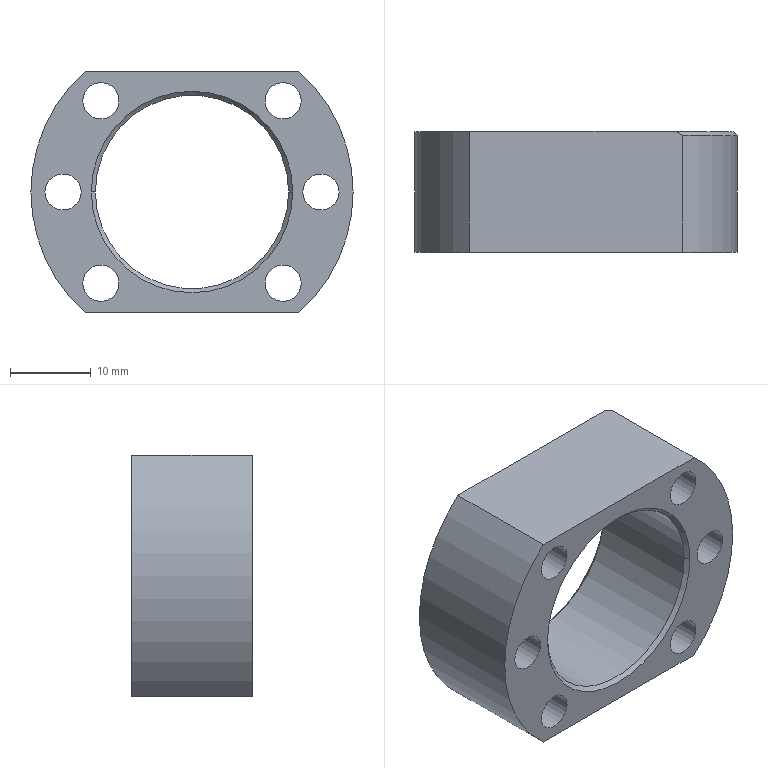Component | SolidWorks | F01AE00111-A2085-1 | 1 solid | 27 faces | box 40 x 15 x 30 mm | volume 7889 mm3 | cylinder 17 | cone 6 | plane 4 | commonest cylinder face diameters 4.5 x12 40 x3 24 x2 | material 6061 Alloy
build123d program:
from build123d import *

# Parameters (mm, degrees)
SKETCH1_R                  = 20
SKETCH1_R_2                = 12
BOSS_EXTRUDE1_DEPTH        = 15
CUT_EXTRUDE1_DEPTH         = 33.016
CHAMFER1_SIZE              = 0.5
F_4_5_4_5_DIAMETER_HOLE1_D = 4.5


with BuildPart() as part:
    # Sketch1 → Boss-Extrude1 (new body)
    with BuildSketch(Plane(origin=(0, 0, 0), x_dir=(1, 0, 0), z_dir=(0, 1, 0))):
        with Locations(Location((0, 0, 0), (0, 0, 270))):
            Circle(SKETCH1_R)
        with Locations(Location((0, 0, 0), (0, 0, 270))):
            Circle(SKETCH1_R_2, mode=Mode.SUBTRACT)
    extrude(amount=BOSS_EXTRUDE1_DEPTH)

    # Sketch2 → Cut-Extrude1 (cut, symmetric)
    with BuildSketch(Plane(origin=(0, 15, 0), x_dir=(1, 0, 0), z_dir=(0, 1, 0))):
        Polygon((15, 119.751), (15, 13.229), (15, -13.229), (15, -119.751), (228.045, -119.751), (228.045, 119.751), align=None)
    cut_extrude1 = extrude(amount=CUT_EXTRUDE1_DEPTH, both=True, mode=Mode.SUBTRACT)

    # Mirror1: Cut-Extrude1 across plane
    add(cut_extrude1.mirror(Plane(origin=(0, 0, 0), x_dir=(0, 0, 1), z_dir=(1, 0, 0))), mode=Mode.SUBTRACT)

    # Chamfer1
    chamfer1_edges = [part.edges().sort_by_distance(p)[0] for p in [
        (0, 0, -12),
        (0, 15, -12),
        (0, 15, -20),
    ]]
    chamfer(chamfer1_edges, length=CHAMFER1_SIZE)

    # 4.5 _4.5_ Diameter Hole1 (through all)
    with Locations(Plane(origin=(0, 15, 0), x_dir=(1, 0, 0), z_dir=(0, 1, 0))):
        with Locations((-11.314, 11.314), (0, 16), (11.314, 11.314), (-11.314, -11.314), (0, -16), (11.314, -11.314)):
            Hole(F_4_5_4_5_DIAMETER_HOLE1_D / 2)


solid = part.part

# Placed as in the assembly
solid = solid.moved(Location((-109.352, -190.452, -272.475), (0, -90, 0)))
STEP:
#1=CARTESIAN_POINT('',(-3.771,-7.498,-11.173));
#2=VERTEX_POINT('',#1);
#3=CARTESIAN_POINT('',(-3.948,-7.498,-11.173));
#4=VERTEX_POINT('',#3);
#5=CARTESIAN_POINT('',(-3.86,-7.498,-11.173));
#6=DIRECTION('',(-0.,1.,0.));
#7=DIRECTION('',(-1.,0.,0.));
#8=AXIS2_PLACEMENT_3D('',#5,#6,#7);
#9=CIRCLE('',#8,0.08858);
#10=EDGE_CURVE('',#2,#4,#9,.T.);
#11=ORIENTED_EDGE('',*,*,#10,.F.);
#12=CARTESIAN_POINT('',(-3.771,-6.908,-11.173));
#13=VERTEX_POINT('',#12);
#14=CARTESIAN_POINT('',(-3.771,-6.908,-11.173));
#15=DIRECTION('',(-0.,1.,0.));
#16=VECTOR('',#15,39.37);
#17=LINE('',#14,#16);
#18=EDGE_CURVE('',#2,#13,#17,.T.);
#19=ORIENTED_EDGE('',*,*,#18,.T.);
#20=CARTESIAN_POINT('',(-3.948,-6.908,-11.173));
#21=VERTEX_POINT('',#20);
#22=CARTESIAN_POINT('',(-3.86,-6.908,-11.173));
#23=DIRECTION('',(-0.,1.,0.));
#24=DIRECTION('',(-1.,0.,0.));
#25=AXIS2_PLACEMENT_3D('',#22,#23,#24);
#26=CIRCLE('',#25,0.08858);
#27=EDGE_CURVE('',#13,#21,#26,.T.);
#28=ORIENTED_EDGE('',*,*,#27,.T.);
#29=CARTESIAN_POINT('',(-3.948,-6.908,-11.173));
#30=DIRECTION('',(-0.,1.,0.));
#31=VECTOR('',#30,39.37);
#32=LINE('',#29,#31);
#33=EDGE_CURVE('',#4,#21,#32,.T.);
#34=ORIENTED_EDGE('',*,*,#33,.F.);
#35=EDGE_LOOP('',(#11,#19,#28,#34));
#36=FACE_OUTER_BOUND('',#35,.T.);
#37=CARTESIAN_POINT('',(-3.86,-6.908,-11.173));
#38=DIRECTION('',(-0.,1.,0.));
#39=DIRECTION('',(-1.,0.,0.));
#40=AXIS2_PLACEMENT_3D('',#37,#38,#39);
#41=CYLINDRICAL_SURFACE('',#40,0.08858);
#42=ADVANCED_FACE('',(#36),#41,.F.);
#43=CARTESIAN_POINT('',(-3.587,-7.498,-10.727));
#44=VERTEX_POINT('',#43);
#45=CARTESIAN_POINT('',(-3.764,-7.498,-10.727));
#46=VERTEX_POINT('',#45);
#47=CARTESIAN_POINT('',(-3.675,-7.498,-10.727));
#48=DIRECTION('',(-0.,1.,0.));
#49=DIRECTION('',(-1.,0.,0.));
#50=AXIS2_PLACEMENT_3D('',#47,#48,#49);
#51=CIRCLE('',#50,0.08858);
#52=EDGE_CURVE('',#44,#46,#51,.T.);
#53=ORIENTED_EDGE('',*,*,#52,.F.);
#54=CARTESIAN_POINT('',(-3.587,-6.908,-10.727));
#55=VERTEX_POINT('',#54);
#56=CARTESIAN_POINT('',(-3.587,-6.908,-10.727));
#57=DIRECTION('',(-0.,1.,0.));
#58=VECTOR('',#57,39.37);
#59=LINE('',#56,#58);
#60=EDGE_CURVE('',#44,#55,#59,.T.);
#61=ORIENTED_EDGE('',*,*,#60,.T.);
#62=CARTESIAN_POINT('',(-3.764,-6.908,-10.727));
#63=VERTEX_POINT('',#62);
#64=CARTESIAN_POINT('',(-3.675,-6.908,-10.727));
#65=DIRECTION('',(-0.,1.,0.));
#66=DIRECTION('',(-1.,0.,0.));
#67=AXIS2_PLACEMENT_3D('',#64,#65,#66);
#68=CIRCLE('',#67,0.08858);
#69=EDGE_CURVE('',#55,#63,#68,.T.);
#70=ORIENTED_EDGE('',*,*,#69,.T.);
#71=CARTESIAN_POINT('',(-3.764,-6.908,-10.727));
#72=DIRECTION('',(-0.,1.,0.));
#73=VECTOR('',#72,39.37);
#74=LINE('',#71,#73);
#75=EDGE_CURVE('',#46,#63,#74,.T.);
#76=ORIENTED_EDGE('',*,*,#75,.F.);
#77=EDGE_LOOP('',(#53,#61,#70,#76));
#78=FACE_OUTER_BOUND('',#77,.T.);
#79=CARTESIAN_POINT('',(-3.675,-6.908,-10.727));
#80=DIRECTION('',(-0.,1.,0.));
#81=DIRECTION('',(-1.,0.,0.));
#82=AXIS2_PLACEMENT_3D('',#79,#80,#81);
#83=CYLINDRICAL_SURFACE('',#82,0.08858);
#84=ADVANCED_FACE('',(#78),#83,.F.);
#85=CARTESIAN_POINT('',(-3.771,-7.498,-10.282));
#86=VERTEX_POINT('',#85);
#87=CARTESIAN_POINT('',(-3.948,-7.498,-10.282));
#88=VERTEX_POINT('',#87);
#89=CARTESIAN_POINT('',(-3.86,-7.498,-10.282));
#90=DIRECTION('',(-0.,1.,0.));
#91=DIRECTION('',(-1.,0.,0.));
#92=AXIS2_PLACEMENT_3D('',#89,#90,#91);
#93=CIRCLE('',#92,0.08858);
#94=EDGE_CURVE('',#86,#88,#93,.T.);
#95=ORIENTED_EDGE('',*,*,#94,.F.);
#96=CARTESIAN_POINT('',(-3.771,-6.908,-10.282));
#97=VERTEX_POINT('',#96);
#98=CARTESIAN_POINT('',(-3.771,-6.908,-10.282));
#99=DIRECTION('',(-0.,1.,0.));
#100=VECTOR('',#99,39.37);
#101=LINE('',#98,#100);
#102=EDGE_CURVE('',#86,#97,#101,.T.);
#103=ORIENTED_EDGE('',*,*,#102,.T.);
#104=CARTESIAN_POINT('',(-3.948,-6.908,-10.282));
#105=VERTEX_POINT('',#104);
#106=CARTESIAN_POINT('',(-3.86,-6.908,-10.282));
#107=DIRECTION('',(-0.,1.,0.));
#108=DIRECTION('',(-1.,0.,0.));
#109=AXIS2_PLACEMENT_3D('',#106,#107,#108);
#110=CIRCLE('',#109,0.08858);
#111=EDGE_CURVE('',#97,#105,#110,.T.);
#112=ORIENTED_EDGE('',*,*,#111,.T.);
#113=CARTESIAN_POINT('',(-3.948,-6.908,-10.282));
#114=DIRECTION('',(-0.,1.,0.));
#115=VECTOR('',#114,39.37);
#116=LINE('',#113,#115);
#117=EDGE_CURVE('',#88,#105,#116,.T.);
#118=ORIENTED_EDGE('',*,*,#117,.F.);
#119=EDGE_LOOP('',(#95,#103,#112,#118));
#120=FACE_OUTER_BOUND('',#119,.T.);
#121=CARTESIAN_POINT('',(-3.86,-6.908,-10.282));
#122=DIRECTION('',(-0.,1.,0.));
#123=DIRECTION('',(-1.,0.,0.));
#124=AXIS2_PLACEMENT_3D('',#121,#122,#123);
#125=CYLINDRICAL_SURFACE('',#124,0.08858);
#126=ADVANCED_FACE('',(#120),#125,.F.);
#127=CARTESIAN_POINT('',(-4.662,-7.498,-11.173));
#128=VERTEX_POINT('',#127);
#129=CARTESIAN_POINT('',(-4.839,-7.498,-11.173));
#130=VERTEX_POINT('',#129);
#131=CARTESIAN_POINT('',(-4.751,-7.498,-11.173));
#132=DIRECTION('',(-0.,1.,0.));
#133=DIRECTION('',(-1.,0.,0.));
#134=AXIS2_PLACEMENT_3D('',#131,#132,#133);
#135=CIRCLE('',#134,0.08858);
#136=EDGE_CURVE('',#128,#130,#135,.T.);
#137=ORIENTED_EDGE('',*,*,#136,.F.);
#138=CARTESIAN_POINT('',(-4.662,-6.908,-11.173));
#139=VERTEX_POINT('',#138);
#140=CARTESIAN_POINT('',(-4.662,-6.908,-11.173));
#141=DIRECTION('',(-0.,1.,0.));
#142=VECTOR('',#141,39.37);
#143=LINE('',#140,#142);
#144=EDGE_CURVE('',#128,#139,#143,.T.);
#145=ORIENTED_EDGE('',*,*,#144,.T.);
#146=CARTESIAN_POINT('',(-4.839,-6.908,-11.173));
#147=VERTEX_POINT('',#146);
#148=CARTESIAN_POINT('',(-4.751,-6.908,-11.173));
#149=DIRECTION('',(-0.,1.,0.));
#150=DIRECTION('',(-1.,0.,0.));
#151=AXIS2_PLACEMENT_3D('',#148,#149,#150);
#152=CIRCLE('',#151,0.08858);
#153=EDGE_CURVE('',#139,#147,#152,.T.);
#154=ORIENTED_EDGE('',*,*,#153,.T.);
#155=CARTESIAN_POINT('',(-4.839,-6.908,-11.173));
#156=DIRECTION('',(-0.,1.,0.));
#157=VECTOR('',#156,39.37);
#158=LINE('',#155,#157);
#159=EDGE_CURVE('',#130,#147,#158,.T.);
#160=ORIENTED_EDGE('',*,*,#159,.F.);
#161=EDGE_LOOP('',(#137,#145,#154,#160));
#162=FACE_OUTER_BOUND('',#161,.T.);
#163=CARTESIAN_POINT('',(-4.751,-6.908,-11.173));
#164=DIRECTION('',(-0.,1.,0.));
#165=DIRECTION('',(-1.,0.,0.));
#166=AXIS2_PLACEMENT_3D('',#163,#164,#165);
#167=CYLINDRICAL_SURFACE('',#166,0.08858);
#168=ADVANCED_FACE('',(#162),#167,.F.);
#169=CARTESIAN_POINT('',(-4.847,-7.498,-10.727));
#170=VERTEX_POINT('',#169);
#171=CARTESIAN_POINT('',(-5.024,-7.498,-10.727));
#172=VERTEX_POINT('',#171);
#173=CARTESIAN_POINT('',(-4.935,-7.498,-10.727));
#174=DIRECTION('',(-0.,1.,0.));
#175=DIRECTION('',(-1.,0.,0.));
#176=AXIS2_PLACEMENT_3D('',#173,#174,#175);
#177=CIRCLE('',#176,0.08858);
#178=EDGE_CURVE('',#170,#172,#177,.T.);
#179=ORIENTED_EDGE('',*,*,#178,.F.);
#180=CARTESIAN_POINT('',(-4.847,-6.908,-10.727));
#181=VERTEX_POINT('',#180);
#182=CARTESIAN_POINT('',(-4.847,-6.908,-10.727));
#183=DIRECTION('',(-0.,1.,0.));
#184=VECTOR('',#183,39.37);
#185=LINE('',#182,#184);
#186=EDGE_CURVE('',#170,#181,#185,.T.);
#187=ORIENTED_EDGE('',*,*,#186,.T.);
#188=CARTESIAN_POINT('',(-5.024,-6.908,-10.727));
#189=VERTEX_POINT('',#188);
#190=CARTESIAN_POINT('',(-4.935,-6.908,-10.727));
#191=DIRECTION('',(-0.,1.,0.));
#192=DIRECTION('',(-1.,0.,0.));
#193=AXIS2_PLACEMENT_3D('',#190,#191,#192);
#194=CIRCLE('',#193,0.08858);
#195=EDGE_CURVE('',#181,#189,#194,.T.);
#196=ORIENTED_EDGE('',*,*,#195,.T.);
#197=CARTESIAN_POINT('',(-5.024,-6.908,-10.727));
#198=DIRECTION('',(-0.,1.,0.));
#199=VECTOR('',#198,39.37);
#200=LINE('',#197,#199);
#201=EDGE_CURVE('',#172,#189,#200,.T.);
#202=ORIENTED_EDGE('',*,*,#201,.F.);
#203=EDGE_LOOP('',(#179,#187,#196,#202));
#204=FACE_OUTER_BOUND('',#203,.T.);
#205=CARTESIAN_POINT('',(-4.935,-6.908,-10.727));
#206=DIRECTION('',(-0.,1.,0.));
#207=DIRECTION('',(-1.,0.,0.));
#208=AXIS2_PLACEMENT_3D('',#205,#206,#207);
#209=CYLINDRICAL_SURFACE('',#208,0.08858);
#210=ADVANCED_FACE('',(#204),#209,.F.);
#211=CARTESIAN_POINT('',(-4.662,-7.498,-10.282));
#212=VERTEX_POINT('',#211);
#213=CARTESIAN_POINT('',(-4.839,-7.498,-10.282));
#214=VERTEX_POINT('',#213);
#215=CARTESIAN_POINT('',(-4.751,-7.498,-10.282));
#216=DIRECTION('',(-0.,1.,0.));
#217=DIRECTION('',(-1.,0.,0.));
#218=AXIS2_PLACEMENT_3D('',#215,#216,#217);
#219=CIRCLE('',#218,0.08858);
#220=EDGE_CURVE('',#212,#214,#219,.T.);
#221=ORIENTED_EDGE('',*,*,#220,.F.);
#222=CARTESIAN_POINT('',(-4.662,-6.908,-10.282));
#223=VERTEX_POINT('',#222);
#224=CARTESIAN_POINT('',(-4.662,-6.908,-10.282));
#225=DIRECTION('',(-0.,1.,0.));
#226=VECTOR('',#225,39.37);
#227=LINE('',#224,#226);
#228=EDGE_CURVE('',#212,#223,#227,.T.);
#229=ORIENTED_EDGE('',*,*,#228,.T.);
#230=CARTESIAN_POINT('',(-4.839,-6.908,-10.282));
#231=VERTEX_POINT('',#230);
#232=CARTESIAN_POINT('',(-4.751,-6.908,-10.282));
#233=DIRECTION('',(-0.,1.,0.));
#234=DIRECTION('',(-1.,0.,0.));
#235=AXIS2_PLACEMENT_3D('',#232,#233,#234);
#236=CIRCLE('',#235,0.08858);
#237=EDGE_CURVE('',#223,#231,#236,.T.);
#238=ORIENTED_EDGE('',*,*,#237,.T.);
#239=CARTESIAN_POINT('',(-4.839,-6.908,-10.282));
#240=DIRECTION('',(-0.,1.,0.));
#241=VECTOR('',#240,39.37);
#242=LINE('',#239,#241);
#243=EDGE_CURVE('',#214,#231,#242,.T.);
#244=ORIENTED_EDGE('',*,*,#243,.F.);
#245=EDGE_LOOP('',(#221,#229,#238,#244));
#246=FACE_OUTER_BOUND('',#245,.T.);
#247=CARTESIAN_POINT('',(-4.751,-6.908,-10.282));
#248=DIRECTION('',(-0.,1.,0.));
#249=DIRECTION('',(-1.,0.,0.));
#250=AXIS2_PLACEMENT_3D('',#247,#248,#249);
#251=CYLINDRICAL_SURFACE('',#250,0.08858);
#252=ADVANCED_FACE('',(#246),#251,.F.);
#253=CARTESIAN_POINT('',(-3.833,-6.927,-10.727));
#254=VERTEX_POINT('',#253);
#255=CARTESIAN_POINT('',(-4.778,-6.927,-10.727));
#256=VERTEX_POINT('',#255);
#257=CARTESIAN_POINT('',(-4.305,-6.927,-10.727));
#258=DIRECTION('',(-0.,1.,0.));
#259=DIRECTION('',(-1.,0.,0.));
#260=AXIS2_PLACEMENT_3D('',#257,#258,#259);
#261=CIRCLE('',#260,0.4724);
#262=EDGE_CURVE('',#254,#256,#261,.T.);
#263=ORIENTED_EDGE('',*,*,#262,.F.);
#264=CARTESIAN_POINT('',(-3.813,-6.908,-10.727));
#265=VERTEX_POINT('',#264);
#266=CARTESIAN_POINT('',(-3.833,-6.927,-10.727));
#267=DIRECTION('',(0.7071,0.7071,-0.));
#268=VECTOR('',#267,39.37);
#269=LINE('',#266,#268);
#270=EDGE_CURVE('',#254,#265,#269,.T.);
#271=ORIENTED_EDGE('',*,*,#270,.T.);
#272=CARTESIAN_POINT('',(-4.797,-6.908,-10.727));
#273=VERTEX_POINT('',#272);
#274=CARTESIAN_POINT('',(-4.305,-6.908,-10.727));
#275=DIRECTION('',(0.,-1.,-0.));
#276=DIRECTION('',(-1.,0.,0.));
#277=AXIS2_PLACEMENT_3D('',#274,#275,#276);
#278=CIRCLE('',#277,0.4921);
#279=EDGE_CURVE('',#273,#265,#278,.T.);
#280=ORIENTED_EDGE('',*,*,#279,.F.);
#281=CARTESIAN_POINT('',(-4.778,-6.927,-10.727));
#282=DIRECTION('',(-0.7071,0.7071,0.));
#283=VECTOR('',#282,39.37);
#284=LINE('',#281,#283);
#285=EDGE_CURVE('',#256,#273,#284,.T.);
#286=ORIENTED_EDGE('',*,*,#285,.F.);
#287=EDGE_LOOP('',(#263,#271,#280,#286));
#288=FACE_OUTER_BOUND('',#287,.T.);
#289=CARTESIAN_POINT('',(-4.305,-6.927,-10.727));
#290=DIRECTION('',(-0.,1.,0.));
#291=DIRECTION('',(-1.,0.,0.));
#292=AXIS2_PLACEMENT_3D('',#289,#290,#291);
#293=CONICAL_SURFACE('',#292,0.4724,0.7854);
#294=ADVANCED_FACE('',(#288),#293,.F.);
#295=CARTESIAN_POINT('',(-3.537,-6.908,-10.727));
#296=VERTEX_POINT('',#295);
#297=CARTESIAN_POINT('',(-3.815,-6.908,-11.318));
#298=VERTEX_POINT('',#297);
#299=CARTESIAN_POINT('',(-4.305,-6.908,-10.727));
#300=DIRECTION('',(-0.,1.,0.));
#301=DIRECTION('',(-1.,0.,0.));
#302=AXIS2_PLACEMENT_3D('',#299,#300,#301);
#303=CIRCLE('',#302,0.7677);
#304=EDGE_CURVE('',#296,#298,#303,.T.);
#305=ORIENTED_EDGE('',*,*,#304,.F.);
#306=CARTESIAN_POINT('',(-3.518,-6.927,-10.727));
#307=VERTEX_POINT('',#306);
#308=CARTESIAN_POINT('',(-3.537,-6.908,-10.727));
#309=DIRECTION('',(0.7071,-0.7071,-0.));
#310=VECTOR('',#309,39.37);
#311=LINE('',#308,#310);
#312=EDGE_CURVE('',#296,#307,#311,.T.);
#313=ORIENTED_EDGE('',*,*,#312,.T.);
#314=CARTESIAN_POINT('',(-3.784,-6.927,-11.318));
#315=VERTEX_POINT('',#314);
#316=CARTESIAN_POINT('',(-4.305,-6.927,-10.727));
#317=DIRECTION('',(0.,-1.,-0.));
#318=DIRECTION('',(-1.,0.,0.));
#319=AXIS2_PLACEMENT_3D('',#316,#317,#318);
#320=CIRCLE('',#319,0.7874);
#321=EDGE_CURVE('',#315,#307,#320,.T.);
#322=ORIENTED_EDGE('',*,*,#321,.F.);
#323=CARTESIAN_POINT('',(-3.815,-6.908,-11.318));
#324=CARTESIAN_POINT('',(-3.805,-6.914,-11.318));
#325=CARTESIAN_POINT('',(-3.794,-6.921,-11.318));
#326=CARTESIAN_POINT('',(-3.784,-6.927,-11.318));
#327=B_SPLINE_CURVE_WITH_KNOTS('',3,(#323,#324,#325,#326),.UNSPECIFIED.,.F.,.F.,(4,4),(0.,0.0009171),.UNSPECIFIED.);
#328=EDGE_CURVE('',#298,#315,#327,.T.);
#329=ORIENTED_EDGE('',*,*,#328,.F.);
#330=EDGE_LOOP('',(#305,#313,#322,#329));
#331=FACE_OUTER_BOUND('',#330,.T.);
#332=CARTESIAN_POINT('',(-4.305,-6.908,-10.727));
#333=DIRECTION('',(0.,-1.,-0.));
#334=DIRECTION('',(1.,0.,-0.));
#335=AXIS2_PLACEMENT_3D('',#332,#333,#334);
#336=CONICAL_SURFACE('',#335,0.7677,0.7854);
#337=ADVANCED_FACE('',(#331),#336,.T.);
#338=CARTESIAN_POINT('',(-4.778,-7.478,-10.727));
#339=VERTEX_POINT('',#338);
#340=CARTESIAN_POINT('',(-3.833,-7.478,-10.727));
#341=VERTEX_POINT('',#340);
#342=CARTESIAN_POINT('',(-4.305,-7.478,-10.727));
#343=DIRECTION('',(0.,-1.,-0.));
#344=DIRECTION('',(-1.,0.,0.));
#345=AXIS2_PLACEMENT_3D('',#342,#343,#344);
#346=CIRCLE('',#345,0.4724);
#347=EDGE_CURVE('',#339,#341,#346,.T.);
#348=ORIENTED_EDGE('',*,*,#347,.F.);
#349=CARTESIAN_POINT('',(-4.797,-7.498,-10.727));
#350=VERTEX_POINT('',#349);
#351=CARTESIAN_POINT('',(-4.797,-7.498,-10.727));
#352=DIRECTION('',(-0.7071,-0.7071,0.));
#353=VECTOR('',#352,39.37);
#354=LINE('',#351,#353);
#355=EDGE_CURVE('',#339,#350,#354,.T.);
#356=ORIENTED_EDGE('',*,*,#355,.T.);
#357=CARTESIAN_POINT('',(-3.813,-7.498,-10.727));
#358=VERTEX_POINT('',#357);
#359=CARTESIAN_POINT('',(-4.305,-7.498,-10.727));
#360=DIRECTION('',(-0.,1.,0.));
#361=DIRECTION('',(-1.,0.,0.));
#362=AXIS2_PLACEMENT_3D('',#359,#360,#361);
#363=CIRCLE('',#362,0.4921);
#364=EDGE_CURVE('',#358,#350,#363,.T.);
#365=ORIENTED_EDGE('',*,*,#364,.F.);
#366=CARTESIAN_POINT('',(-3.813,-7.498,-10.727));
#367=DIRECTION('',(0.7071,-0.7071,-0.));
#368=VECTOR('',#367,39.37);
#369=LINE('',#366,#368);
#370=EDGE_CURVE('',#341,#358,#369,.T.);
#371=ORIENTED_EDGE('',*,*,#370,.F.);
#372=EDGE_LOOP('',(#348,#356,#365,#371));
#373=FACE_OUTER_BOUND('',#372,.T.);
#374=CARTESIAN_POINT('',(-4.305,-7.498,-10.727));
#375=DIRECTION('',(0.,-1.,-0.));
#376=DIRECTION('',(1.,0.,-0.));
#377=AXIS2_PLACEMENT_3D('',#374,#375,#376);
#378=CONICAL_SURFACE('',#377,0.4921,0.7854);
#379=ADVANCED_FACE('',(#373),#378,.F.);
#380=ORIENTED_EDGE('',*,*,#262,.T.);
#381=CARTESIAN_POINT('',(-4.778,-6.908,-10.727));
#382=DIRECTION('',(0.,-1.,-0.));
#383=VECTOR('',#382,39.37);
#384=LINE('',#381,#383);
#385=EDGE_CURVE('',#256,#339,#384,.T.);
#386=ORIENTED_EDGE('',*,*,#385,.T.);
#387=ORIENTED_EDGE('',*,*,#347,.T.);
#388=CARTESIAN_POINT('',(-3.833,-6.908,-10.727));
#389=DIRECTION('',(0.,-1.,-0.));
#390=VECTOR('',#389,39.37);
#391=LINE('',#388,#390);
#392=EDGE_CURVE('',#254,#341,#391,.T.);
#393=ORIENTED_EDGE('',*,*,#392,.F.);
#394=EDGE_LOOP('',(#380,#386,#387,#393));
#395=FACE_OUTER_BOUND('',#394,.T.);
#396=CARTESIAN_POINT('',(-4.305,-6.908,-10.727));
#397=DIRECTION('',(0.,-1.,-0.));
#398=DIRECTION('',(1.,0.,-0.));
#399=AXIS2_PLACEMENT_3D('',#396,#397,#398);
#400=CYLINDRICAL_SURFACE('',#399,0.4724);
#401=ADVANCED_FACE('',(#395),#400,.F.);
#402=ORIENTED_EDGE('',*,*,#321,.T.);
#403=CARTESIAN_POINT('',(-3.518,-7.498,-10.727));
#404=VERTEX_POINT('',#403);
#405=CARTESIAN_POINT('',(-3.518,-6.908,-10.727));
#406=DIRECTION('',(0.,-1.,-0.));
#407=VECTOR('',#406,39.37);
#408=LINE('',#405,#407);
#409=EDGE_CURVE('',#307,#404,#408,.T.);
#410=ORIENTED_EDGE('',*,*,#409,.T.);
#411=CARTESIAN_POINT('',(-3.784,-7.498,-11.318));
#412=VERTEX_POINT('',#411);
#413=CARTESIAN_POINT('',(-4.305,-7.498,-10.727));
#414=DIRECTION('',(-0.,1.,0.));
#415=DIRECTION('',(-1.,0.,0.));
#416=AXIS2_PLACEMENT_3D('',#413,#414,#415);
#417=CIRCLE('',#416,0.7874);
#418=EDGE_CURVE('',#404,#412,#417,.T.);
#419=ORIENTED_EDGE('',*,*,#418,.T.);
#420=CARTESIAN_POINT('',(-3.784,-6.908,-11.318));
#421=DIRECTION('',(-0.,1.,0.));
#422=VECTOR('',#421,39.37);
#423=LINE('',#420,#422);
#424=EDGE_CURVE('',#412,#315,#423,.T.);
#425=ORIENTED_EDGE('',*,*,#424,.T.);
#426=EDGE_LOOP('',(#402,#410,#419,#425));
#427=FACE_OUTER_BOUND('',#426,.T.);
#428=CARTESIAN_POINT('',(-4.305,-6.908,-10.727));
#429=DIRECTION('',(0.,-1.,-0.));
#430=DIRECTION('',(1.,0.,-0.));
#431=AXIS2_PLACEMENT_3D('',#428,#429,#430);
#432=CYLINDRICAL_SURFACE('',#431,0.7874);
#433=ADVANCED_FACE('',(#427),#432,.T.);
#434=CARTESIAN_POINT('',(-4.826,-6.908,-11.318));
#435=VERTEX_POINT('',#434);
#436=CARTESIAN_POINT('',(-4.826,-6.908,-10.137));
#437=VERTEX_POINT('',#436);
#438=CARTESIAN_POINT('',(-4.305,-6.908,-10.727));
#439=DIRECTION('',(-0.,1.,0.));
#440=DIRECTION('',(-1.,0.,0.));
#441=AXIS2_PLACEMENT_3D('',#438,#439,#440);
#442=CIRCLE('',#441,0.7874);
#443=EDGE_CURVE('',#435,#437,#442,.T.);
#444=ORIENTED_EDGE('',*,*,#443,.F.);
#445=CARTESIAN_POINT('',(-4.826,-7.498,-11.318));
#446=VERTEX_POINT('',#445);
#447=CARTESIAN_POINT('',(-4.826,-6.908,-11.318));
#448=DIRECTION('',(0.,-1.,-0.));
#449=VECTOR('',#448,39.37);
#450=LINE('',#447,#449);
#451=EDGE_CURVE('',#435,#446,#450,.T.);
#452=ORIENTED_EDGE('',*,*,#451,.T.);
#453=CARTESIAN_POINT('',(-4.826,-7.498,-10.137));
#454=VERTEX_POINT('',#453);
#455=CARTESIAN_POINT('',(-4.305,-7.498,-10.727));
#456=DIRECTION('',(-0.,1.,0.));
#457=DIRECTION('',(-1.,0.,0.));
#458=AXIS2_PLACEMENT_3D('',#455,#456,#457);
#459=CIRCLE('',#458,0.7874);
#460=EDGE_CURVE('',#446,#454,#459,.T.);
#461=ORIENTED_EDGE('',*,*,#460,.T.);
#462=CARTESIAN_POINT('',(-4.826,-6.908,-10.137));
#463=DIRECTION('',(0.,-1.,-0.));
#464=VECTOR('',#463,39.37);
#465=LINE('',#462,#464);
#466=EDGE_CURVE('',#437,#454,#465,.T.);
#467=ORIENTED_EDGE('',*,*,#466,.F.);
#468=EDGE_LOOP('',(#444,#452,#461,#467));
#469=FACE_OUTER_BOUND('',#468,.T.);
#470=CARTESIAN_POINT('',(-4.305,-6.908,-10.727));
#471=DIRECTION('',(0.,-1.,-0.));
#472=DIRECTION('',(1.,0.,-0.));
#473=AXIS2_PLACEMENT_3D('',#470,#471,#472);
#474=CYLINDRICAL_SURFACE('',#473,0.7874);
#475=ADVANCED_FACE('',(#469),#474,.T.);
#476=CARTESIAN_POINT('',(-3.86,-6.908,-11.173));
#477=DIRECTION('',(-0.,1.,0.));
#478=DIRECTION('',(-1.,0.,0.));
#479=AXIS2_PLACEMENT_3D('',#476,#477,#478);
#480=CIRCLE('',#479,0.08858);
#481=EDGE_CURVE('',#21,#13,#480,.T.);
#482=ORIENTED_EDGE('',*,*,#481,.F.);
#483=ORIENTED_EDGE('',*,*,#27,.F.);
#484=EDGE_LOOP('',(#482,#483));
#485=FACE_BOUND('',#484,.T.);
#486=CARTESIAN_POINT('',(-3.675,-6.908,-10.727));
#487=DIRECTION('',(-0.,1.,0.));
#488=DIRECTION('',(-1.,0.,0.));
#489=AXIS2_PLACEMENT_3D('',#486,#487,#488);
#490=CIRCLE('',#489,0.08858);
#491=EDGE_CURVE('',#63,#55,#490,.T.);
#492=ORIENTED_EDGE('',*,*,#491,.F.);
#493=ORIENTED_EDGE('',*,*,#69,.F.);
#494=EDGE_LOOP('',(#492,#493));
#495=FACE_BOUND('',#494,.T.);
#496=CARTESIAN_POINT('',(-3.86,-6.908,-10.282));
#497=DIRECTION('',(-0.,1.,0.));
#498=DIRECTION('',(-1.,0.,0.));
#499=AXIS2_PLACEMENT_3D('',#496,#497,#498);
#500=CIRCLE('',#499,0.08858);
#501=EDGE_CURVE('',#105,#97,#500,.T.);
#502=ORIENTED_EDGE('',*,*,#501,.F.);
#503=ORIENTED_EDGE('',*,*,#111,.F.);
#504=EDGE_LOOP('',(#502,#503));
#505=FACE_BOUND('',#504,.T.);
#506=CARTESIAN_POINT('',(-4.751,-6.908,-11.173));
#507=DIRECTION('',(-0.,1.,0.));
#508=DIRECTION('',(-1.,0.,0.));
#509=AXIS2_PLACEMENT_3D('',#506,#507,#508);
#510=CIRCLE('',#509,0.08858);
#511=EDGE_CURVE('',#147,#139,#510,.T.);
#512=ORIENTED_EDGE('',*,*,#511,.F.);
#513=ORIENTED_EDGE('',*,*,#153,.F.);
#514=EDGE_LOOP('',(#512,#513));
#515=FACE_BOUND('',#514,.T.);
#516=CARTESIAN_POINT('',(-4.935,-6.908,-10.727));
#517=DIRECTION('',(-0.,1.,0.));
#518=DIRECTION('',(-1.,0.,0.));
#519=AXIS2_PLACEMENT_3D('',#516,#517,#518);
#520=CIRCLE('',#519,0.08858);
#521=EDGE_CURVE('',#189,#181,#520,.T.);
#522=ORIENTED_EDGE('',*,*,#521,.F.);
#523=ORIENTED_EDGE('',*,*,#195,.F.);
#524=EDGE_LOOP('',(#522,#523));
#525=FACE_BOUND('',#524,.T.);
#526=CARTESIAN_POINT('',(-4.751,-6.908,-10.282));
#527=DIRECTION('',(-0.,1.,0.));
#528=DIRECTION('',(-1.,0.,0.));
#529=AXIS2_PLACEMENT_3D('',#526,#527,#528);
#530=CIRCLE('',#529,0.08858);
#531=EDGE_CURVE('',#231,#223,#530,.T.);
#532=ORIENTED_EDGE('',*,*,#531,.F.);
#533=ORIENTED_EDGE('',*,*,#237,.F.);
#534=EDGE_LOOP('',(#532,#533));
#535=FACE_BOUND('',#534,.T.);
#536=ORIENTED_EDGE('',*,*,#279,.T.);
#537=CARTESIAN_POINT('',(-4.305,-6.908,-10.727));
#538=DIRECTION('',(0.,-1.,-0.));
#539=DIRECTION('',(-1.,0.,0.));
#540=AXIS2_PLACEMENT_3D('',#537,#538,#539);
#541=CIRCLE('',#540,0.4921);
#542=EDGE_CURVE('',#265,#273,#541,.T.);
#543=ORIENTED_EDGE('',*,*,#542,.T.);
#544=EDGE_LOOP('',(#536,#543));
#545=FACE_BOUND('',#544,.T.);
#546=CARTESIAN_POINT('',(-3.815,-6.908,-10.137));
#547=VERTEX_POINT('',#546);
#548=CARTESIAN_POINT('',(-4.305,-6.908,-10.137));
#549=DIRECTION('',(1.,0.,-0.));
#550=VECTOR('',#549,39.37);
#551=LINE('',#548,#550);
#552=EDGE_CURVE('',#437,#547,#551,.T.);
#553=ORIENTED_EDGE('',*,*,#552,.T.);
#554=CARTESIAN_POINT('',(-4.305,-6.908,-10.727));
#555=DIRECTION('',(-0.,1.,0.));
#556=DIRECTION('',(-1.,0.,0.));
#557=AXIS2_PLACEMENT_3D('',#554,#555,#556);
#558=CIRCLE('',#557,0.7677);
#559=EDGE_CURVE('',#547,#296,#558,.T.);
#560=ORIENTED_EDGE('',*,*,#559,.T.);
#561=ORIENTED_EDGE('',*,*,#304,.T.);
#562=CARTESIAN_POINT('',(-4.305,-6.908,-11.318));
#563=DIRECTION('',(1.,0.,-0.));
#564=VECTOR('',#563,39.37);
#565=LINE('',#562,#564);
#566=EDGE_CURVE('',#435,#298,#565,.T.);
#567=ORIENTED_EDGE('',*,*,#566,.F.);
#568=ORIENTED_EDGE('',*,*,#443,.T.);
#569=EDGE_LOOP('',(#553,#560,#561,#567,#568));
#570=FACE_OUTER_BOUND('',#569,.T.);
#571=CARTESIAN_POINT('',(-4.305,-6.908,-10.727));
#572=DIRECTION('',(-0.,1.,0.));
#573=DIRECTION('',(-1.,-0.,0.));
#574=AXIS2_PLACEMENT_3D('',#571,#572,#573);
#575=PLANE('',#574);
#576=ADVANCED_FACE('',(#485,#495,#505,#515,#525,#535,#545,#570),#575,.T.);
#577=CARTESIAN_POINT('',(-3.86,-7.498,-11.173));
#578=DIRECTION('',(-0.,1.,0.));
#579=DIRECTION('',(-1.,0.,0.));
#580=AXIS2_PLACEMENT_3D('',#577,#578,#579);
#581=CIRCLE('',#580,0.08858);
#582=EDGE_CURVE('',#4,#2,#581,.T.);
#583=ORIENTED_EDGE('',*,*,#582,.T.);
#584=ORIENTED_EDGE('',*,*,#10,.T.);
#585=EDGE_LOOP('',(#583,#584));
#586=FACE_BOUND('',#585,.T.);
#587=CARTESIAN_POINT('',(-3.675,-7.498,-10.727));
#588=DIRECTION('',(-0.,1.,0.));
#589=DIRECTION('',(-1.,0.,0.));
#590=AXIS2_PLACEMENT_3D('',#587,#588,#589);
#591=CIRCLE('',#590,0.08858);
#592=EDGE_CURVE('',#46,#44,#591,.T.);
#593=ORIENTED_EDGE('',*,*,#592,.T.);
#594=ORIENTED_EDGE('',*,*,#52,.T.);
#595=EDGE_LOOP('',(#593,#594));
#596=FACE_BOUND('',#595,.T.);
#597=CARTESIAN_POINT('',(-3.86,-7.498,-10.282));
#598=DIRECTION('',(-0.,1.,0.));
#599=DIRECTION('',(-1.,0.,0.));
#600=AXIS2_PLACEMENT_3D('',#597,#598,#599);
#601=CIRCLE('',#600,0.08858);
#602=EDGE_CURVE('',#88,#86,#601,.T.);
#603=ORIENTED_EDGE('',*,*,#602,.T.);
#604=ORIENTED_EDGE('',*,*,#94,.T.);
#605=EDGE_LOOP('',(#603,#604));
#606=FACE_BOUND('',#605,.T.);
#607=CARTESIAN_POINT('',(-4.751,-7.498,-11.173));
#608=DIRECTION('',(-0.,1.,0.));
#609=DIRECTION('',(-1.,0.,0.));
#610=AXIS2_PLACEMENT_3D('',#607,#608,#609);
#611=CIRCLE('',#610,0.08858);
#612=EDGE_CURVE('',#130,#128,#611,.T.);
#613=ORIENTED_EDGE('',*,*,#612,.T.);
#614=ORIENTED_EDGE('',*,*,#136,.T.);
#615=EDGE_LOOP('',(#613,#614));
#616=FACE_BOUND('',#615,.T.);
#617=CARTESIAN_POINT('',(-4.935,-7.498,-10.727));
#618=DIRECTION('',(-0.,1.,0.));
#619=DIRECTION('',(-1.,0.,0.));
#620=AXIS2_PLACEMENT_3D('',#617,#618,#619);
#621=CIRCLE('',#620,0.08858);
#622=EDGE_CURVE('',#172,#170,#621,.T.);
#623=ORIENTED_EDGE('',*,*,#622,.T.);
#624=ORIENTED_EDGE('',*,*,#178,.T.);
#625=EDGE_LOOP('',(#623,#624));
#626=FACE_BOUND('',#625,.T.);
#627=CARTESIAN_POINT('',(-4.751,-7.498,-10.282));
#628=DIRECTION('',(-0.,1.,0.));
#629=DIRECTION('',(-1.,0.,0.));
#630=AXIS2_PLACEMENT_3D('',#627,#628,#629);
#631=CIRCLE('',#630,0.08858);
#632=EDGE_CURVE('',#214,#212,#631,.T.);
#633=ORIENTED_EDGE('',*,*,#632,.T.);
#634=ORIENTED_EDGE('',*,*,#220,.T.);
#635=EDGE_LOOP('',(#633,#634));
#636=FACE_BOUND('',#635,.T.);
#637=ORIENTED_EDGE('',*,*,#364,.T.);
#638=CARTESIAN_POINT('',(-4.305,-7.498,-10.727));
#639=DIRECTION('',(-0.,1.,0.));
#640=DIRECTION('',(-1.,0.,0.));
#641=AXIS2_PLACEMENT_3D('',#638,#639,#640);
#642=CIRCLE('',#641,0.4921);
#643=EDGE_CURVE('',#350,#358,#642,.T.);
#644=ORIENTED_EDGE('',*,*,#643,.T.);
#645=EDGE_LOOP('',(#637,#644));
#646=FACE_BOUND('',#645,.T.);
#647=ORIENTED_EDGE('',*,*,#460,.F.);
#648=CARTESIAN_POINT('',(-4.305,-7.498,-11.318));
#649=DIRECTION('',(1.,0.,-0.));
#650=VECTOR('',#649,39.37);
#651=LINE('',#648,#650);
#652=EDGE_CURVE('',#446,#412,#651,.T.);
#653=ORIENTED_EDGE('',*,*,#652,.T.);
#654=ORIENTED_EDGE('',*,*,#418,.F.);
#655=CARTESIAN_POINT('',(-3.784,-7.498,-10.137));
#656=VERTEX_POINT('',#655);
#657=CARTESIAN_POINT('',(-4.305,-7.498,-10.727));
#658=DIRECTION('',(-0.,1.,0.));
#659=DIRECTION('',(-1.,0.,0.));
#660=AXIS2_PLACEMENT_3D('',#657,#658,#659);
#661=CIRCLE('',#660,0.7874);
#662=EDGE_CURVE('',#656,#404,#661,.T.);
#663=ORIENTED_EDGE('',*,*,#662,.F.);
#664=CARTESIAN_POINT('',(-4.305,-7.498,-10.137));
#665=DIRECTION('',(1.,0.,-0.));
#666=VECTOR('',#665,39.37);
#667=LINE('',#664,#666);
#668=EDGE_CURVE('',#454,#656,#667,.T.);
#669=ORIENTED_EDGE('',*,*,#668,.F.);
#670=EDGE_LOOP('',(#647,#653,#654,#663,#669));
#671=FACE_OUTER_BOUND('',#670,.T.);
#672=CARTESIAN_POINT('',(-4.305,-7.498,-10.727));
#673=DIRECTION('',(-0.,1.,0.));
#674=DIRECTION('',(-1.,-0.,0.));
#675=AXIS2_PLACEMENT_3D('',#672,#673,#674);
#676=PLANE('',#675);
#677=ADVANCED_FACE('',(#586,#596,#606,#616,#626,#636,#646,#671),#676,.F.);
#678=ORIENTED_EDGE('',*,*,#409,.F.);
#679=CARTESIAN_POINT('',(-3.784,-6.927,-10.137));
#680=VERTEX_POINT('',#679);
#681=CARTESIAN_POINT('',(-4.305,-6.927,-10.727));
#682=DIRECTION('',(0.,-1.,-0.));
#683=DIRECTION('',(-1.,0.,0.));
#684=AXIS2_PLACEMENT_3D('',#681,#682,#683);
#685=CIRCLE('',#684,0.7874);
#686=EDGE_CURVE('',#307,#680,#685,.T.);
#687=ORIENTED_EDGE('',*,*,#686,.T.);
#688=CARTESIAN_POINT('',(-3.784,-6.908,-10.137));
#689=DIRECTION('',(-0.,1.,0.));
#690=VECTOR('',#689,39.37);
#691=LINE('',#688,#690);
#692=EDGE_CURVE('',#656,#680,#691,.T.);
#693=ORIENTED_EDGE('',*,*,#692,.F.);
#694=ORIENTED_EDGE('',*,*,#662,.T.);
#695=EDGE_LOOP('',(#678,#687,#693,#694));
#696=FACE_OUTER_BOUND('',#695,.T.);
#697=CARTESIAN_POINT('',(-4.305,-6.908,-10.727));
#698=DIRECTION('',(0.,-1.,-0.));
#699=DIRECTION('',(1.,0.,-0.));
#700=AXIS2_PLACEMENT_3D('',#697,#698,#699);
#701=CYLINDRICAL_SURFACE('',#700,0.7874);
#702=ADVANCED_FACE('',(#696),#701,.T.);
#703=ORIENTED_EDGE('',*,*,#385,.F.);
#704=CARTESIAN_POINT('',(-4.305,-6.927,-10.727));
#705=DIRECTION('',(-0.,1.,0.));
#706=DIRECTION('',(-1.,0.,0.));
#707=AXIS2_PLACEMENT_3D('',#704,#705,#706);
#708=CIRCLE('',#707,0.4724);
#709=EDGE_CURVE('',#256,#254,#708,.T.);
#710=ORIENTED_EDGE('',*,*,#709,.T.);
#711=ORIENTED_EDGE('',*,*,#392,.T.);
#712=CARTESIAN_POINT('',(-4.305,-7.478,-10.727));
#713=DIRECTION('',(0.,-1.,-0.));
#714=DIRECTION('',(-1.,0.,0.));
#715=AXIS2_PLACEMENT_3D('',#712,#713,#714);
#716=CIRCLE('',#715,0.4724);
#717=EDGE_CURVE('',#341,#339,#716,.T.);
#718=ORIENTED_EDGE('',*,*,#717,.T.);
#719=EDGE_LOOP('',(#703,#710,#711,#718));
#720=FACE_OUTER_BOUND('',#719,.T.);
#721=CARTESIAN_POINT('',(-4.305,-6.908,-10.727));
#722=DIRECTION('',(0.,-1.,-0.));
#723=DIRECTION('',(1.,0.,-0.));
#724=AXIS2_PLACEMENT_3D('',#721,#722,#723);
#725=CYLINDRICAL_SURFACE('',#724,0.4724);
#726=ADVANCED_FACE('',(#720),#725,.F.);
#727=ORIENTED_EDGE('',*,*,#692,.T.);
#728=CARTESIAN_POINT('',(-3.784,-6.927,-10.137));
#729=CARTESIAN_POINT('',(-3.794,-6.921,-10.137));
#730=CARTESIAN_POINT('',(-3.805,-6.914,-10.137));
#731=CARTESIAN_POINT('',(-3.815,-6.908,-10.137));
#732=B_SPLINE_CURVE_WITH_KNOTS('',3,(#728,#729,#730,#731),.UNSPECIFIED.,.F.,.F.,(4,4),(0.,0.0009171),.UNSPECIFIED.);
#733=EDGE_CURVE('',#680,#547,#732,.T.);
#734=ORIENTED_EDGE('',*,*,#733,.T.);
#735=ORIENTED_EDGE('',*,*,#552,.F.);
#736=ORIENTED_EDGE('',*,*,#466,.T.);
#737=ORIENTED_EDGE('',*,*,#668,.T.);
#738=EDGE_LOOP('',(#727,#734,#735,#736,#737));
#739=FACE_OUTER_BOUND('',#738,.T.);
#740=CARTESIAN_POINT('',(-3.784,-4.027,-10.137));
#741=DIRECTION('',(0.,-0.,1.));
#742=DIRECTION('',(1.,0.,-0.));
#743=AXIS2_PLACEMENT_3D('',#740,#741,#742);
#744=PLANE('',#743);
#745=ADVANCED_FACE('',(#739),#744,.T.);
#746=ORIENTED_EDGE('',*,*,#566,.T.);
#747=ORIENTED_EDGE('',*,*,#328,.T.);
#748=ORIENTED_EDGE('',*,*,#424,.F.);
#749=ORIENTED_EDGE('',*,*,#652,.F.);
#750=ORIENTED_EDGE('',*,*,#451,.F.);
#751=EDGE_LOOP('',(#746,#747,#748,#749,#750));
#752=FACE_OUTER_BOUND('',#751,.T.);
#753=CARTESIAN_POINT('',(-3.784,-4.19,-11.318));
#754=DIRECTION('',(0.,-0.,1.));
#755=DIRECTION('',(1.,0.,-0.));
#756=AXIS2_PLACEMENT_3D('',#753,#754,#755);
#757=PLANE('',#756);
#758=ADVANCED_FACE('',(#752),#757,.F.);
#759=ORIENTED_EDGE('',*,*,#355,.F.);
#760=ORIENTED_EDGE('',*,*,#717,.F.);
#761=ORIENTED_EDGE('',*,*,#370,.T.);
#762=ORIENTED_EDGE('',*,*,#643,.F.);
#763=EDGE_LOOP('',(#759,#760,#761,#762));
#764=FACE_OUTER_BOUND('',#763,.T.);
#765=CARTESIAN_POINT('',(-4.305,-7.498,-10.727));
#766=DIRECTION('',(0.,-1.,-0.));
#767=DIRECTION('',(1.,0.,-0.));
#768=AXIS2_PLACEMENT_3D('',#765,#766,#767);
#769=CONICAL_SURFACE('',#768,0.4921,0.7854);
#770=ADVANCED_FACE('',(#764),#769,.F.);
#771=ORIENTED_EDGE('',*,*,#312,.F.);
#772=ORIENTED_EDGE('',*,*,#559,.F.);
#773=ORIENTED_EDGE('',*,*,#733,.F.);
#774=ORIENTED_EDGE('',*,*,#686,.F.);
#775=EDGE_LOOP('',(#771,#772,#773,#774));
#776=FACE_OUTER_BOUND('',#775,.T.);
#777=CARTESIAN_POINT('',(-4.305,-6.908,-10.727));
#778=DIRECTION('',(0.,-1.,-0.));
#779=DIRECTION('',(1.,0.,-0.));
#780=AXIS2_PLACEMENT_3D('',#777,#778,#779);
#781=CONICAL_SURFACE('',#780,0.7677,0.7854);
#782=ADVANCED_FACE('',(#776),#781,.T.);
#783=ORIENTED_EDGE('',*,*,#270,.F.);
#784=ORIENTED_EDGE('',*,*,#709,.F.);
#785=ORIENTED_EDGE('',*,*,#285,.T.);
#786=ORIENTED_EDGE('',*,*,#542,.F.);
#787=EDGE_LOOP('',(#783,#784,#785,#786));
#788=FACE_OUTER_BOUND('',#787,.T.);
#789=CARTESIAN_POINT('',(-4.305,-6.927,-10.727));
#790=DIRECTION('',(-0.,1.,0.));
#791=DIRECTION('',(-1.,0.,0.));
#792=AXIS2_PLACEMENT_3D('',#789,#790,#791);
#793=CONICAL_SURFACE('',#792,0.4724,0.7854);
#794=ADVANCED_FACE('',(#788),#793,.F.);
#795=ORIENTED_EDGE('',*,*,#228,.F.);
#796=ORIENTED_EDGE('',*,*,#632,.F.);
#797=ORIENTED_EDGE('',*,*,#243,.T.);
#798=ORIENTED_EDGE('',*,*,#531,.T.);
#799=EDGE_LOOP('',(#795,#796,#797,#798));
#800=FACE_OUTER_BOUND('',#799,.T.);
#801=CARTESIAN_POINT('',(-4.751,-6.908,-10.282));
#802=DIRECTION('',(-0.,1.,0.));
#803=DIRECTION('',(-1.,0.,0.));
#804=AXIS2_PLACEMENT_3D('',#801,#802,#803);
#805=CYLINDRICAL_SURFACE('',#804,0.08858);
#806=ADVANCED_FACE('',(#800),#805,.F.);
#807=ORIENTED_EDGE('',*,*,#186,.F.);
#808=ORIENTED_EDGE('',*,*,#622,.F.);
#809=ORIENTED_EDGE('',*,*,#201,.T.);
#810=ORIENTED_EDGE('',*,*,#521,.T.);
#811=EDGE_LOOP('',(#807,#808,#809,#810));
#812=FACE_OUTER_BOUND('',#811,.T.);
#813=CARTESIAN_POINT('',(-4.935,-6.908,-10.727));
#814=DIRECTION('',(-0.,1.,0.));
#815=DIRECTION('',(-1.,0.,0.));
#816=AXIS2_PLACEMENT_3D('',#813,#814,#815);
#817=CYLINDRICAL_SURFACE('',#816,0.08858);
#818=ADVANCED_FACE('',(#812),#817,.F.);
#819=ORIENTED_EDGE('',*,*,#144,.F.);
#820=ORIENTED_EDGE('',*,*,#612,.F.);
#821=ORIENTED_EDGE('',*,*,#159,.T.);
#822=ORIENTED_EDGE('',*,*,#511,.T.);
#823=EDGE_LOOP('',(#819,#820,#821,#822));
#824=FACE_OUTER_BOUND('',#823,.T.);
#825=CARTESIAN_POINT('',(-4.751,-6.908,-11.173));
#826=DIRECTION('',(-0.,1.,0.));
#827=DIRECTION('',(-1.,0.,0.));
#828=AXIS2_PLACEMENT_3D('',#825,#826,#827);
#829=CYLINDRICAL_SURFACE('',#828,0.08858);
#830=ADVANCED_FACE('',(#824),#829,.F.);
#831=ORIENTED_EDGE('',*,*,#102,.F.);
#832=ORIENTED_EDGE('',*,*,#602,.F.);
#833=ORIENTED_EDGE('',*,*,#117,.T.);
#834=ORIENTED_EDGE('',*,*,#501,.T.);
#835=EDGE_LOOP('',(#831,#832,#833,#834));
#836=FACE_OUTER_BOUND('',#835,.T.);
#837=CARTESIAN_POINT('',(-3.86,-6.908,-10.282));
#838=DIRECTION('',(-0.,1.,0.));
#839=DIRECTION('',(-1.,0.,0.));
#840=AXIS2_PLACEMENT_3D('',#837,#838,#839);
#841=CYLINDRICAL_SURFACE('',#840,0.08858);
#842=ADVANCED_FACE('',(#836),#841,.F.);
#843=ORIENTED_EDGE('',*,*,#60,.F.);
#844=ORIENTED_EDGE('',*,*,#592,.F.);
#845=ORIENTED_EDGE('',*,*,#75,.T.);
#846=ORIENTED_EDGE('',*,*,#491,.T.);
#847=EDGE_LOOP('',(#843,#844,#845,#846));
#848=FACE_OUTER_BOUND('',#847,.T.);
#849=CARTESIAN_POINT('',(-3.675,-6.908,-10.727));
#850=DIRECTION('',(-0.,1.,0.));
#851=DIRECTION('',(-1.,0.,0.));
#852=AXIS2_PLACEMENT_3D('',#849,#850,#851);
#853=CYLINDRICAL_SURFACE('',#852,0.08858);
#854=ADVANCED_FACE('',(#848),#853,.F.);
#855=ORIENTED_EDGE('',*,*,#18,.F.);
#856=ORIENTED_EDGE('',*,*,#582,.F.);
#857=ORIENTED_EDGE('',*,*,#33,.T.);
#858=ORIENTED_EDGE('',*,*,#481,.T.);
#859=EDGE_LOOP('',(#855,#856,#857,#858));
#860=FACE_OUTER_BOUND('',#859,.T.);
#861=CARTESIAN_POINT('',(-3.86,-6.908,-11.173));
#862=DIRECTION('',(-0.,1.,0.));
#863=DIRECTION('',(-1.,0.,0.));
#864=AXIS2_PLACEMENT_3D('',#861,#862,#863);
#865=CYLINDRICAL_SURFACE('',#864,0.08858);
#866=ADVANCED_FACE('',(#860),#865,.F.);
#867=CLOSED_SHELL('',(#42,#84,#126,#168,#210,#252,#294,#337,#379,#401,#433,#475,#576,#677,#702,#726,#745,#758,#770,#782,#794,#806,#818,#830,#842,#854,#866));
#868=MANIFOLD_SOLID_BREP('',#867);
#869=CARTESIAN_POINT('',(0.,0.,0.));
#870=DIRECTION('',(0.,0.,1.));
#871=DIRECTION('',(1.,0.,0.));
#872=AXIS2_PLACEMENT_3D('',#869,#870,#871);
#873=(LENGTH_UNIT()NAMED_UNIT(*)SI_UNIT($,.METRE.));
#874=LENGTH_MEASURE_WITH_UNIT(LENGTH_MEASURE(0.0254),#873);
#875=DIMENSIONAL_EXPONENTS(1.,0.,0.,0.,0.,0.,0.);
#876=(CONVERSION_BASED_UNIT('',#874)LENGTH_UNIT()NAMED_UNIT(#875));
#877=UNCERTAINTY_MEASURE_WITH_UNIT(LENGTH_MEASURE(0.00001),#876,'','');
#878=(NAMED_UNIT(*)PLANE_ANGLE_UNIT()SI_UNIT($,.RADIAN.));
#879=(NAMED_UNIT(*)SI_UNIT($,.STERADIAN.)SOLID_ANGLE_UNIT());
#880=(GEOMETRIC_REPRESENTATION_CONTEXT(3)GLOBAL_UNCERTAINTY_ASSIGNED_CONTEXT((#877))GLOBAL_UNIT_ASSIGNED_CONTEXT((#876,#878,#879))REPRESENTATION_CONTEXT('',''));
#881=ADVANCED_BREP_SHAPE_REPRESENTATION('',(#868,#872),#880);
#882=COLOUR_RGB('',0.7922,0.8196,0.9333);
#883=FILL_AREA_STYLE_COLOUR('',#882);
#884=FILL_AREA_STYLE('',(#883));
#885=SURFACE_STYLE_FILL_AREA(#884);
#886=SURFACE_SIDE_STYLE('',(#885));
#887=SURFACE_STYLE_USAGE(.BOTH.,#886);
#888=PRESENTATION_STYLE_ASSIGNMENT((#887));
#889=STYLED_ITEM('',(#888),#868);
#890=PRESENTATION_LAYER_ASSIGNMENT('','',(#889));
#891=(LENGTH_UNIT()NAMED_UNIT(*)SI_UNIT($,.METRE.));
#892=LENGTH_MEASURE_WITH_UNIT(LENGTH_MEASURE(0.0254),#891);
#893=DIMENSIONAL_EXPONENTS(1.,0.,0.,0.,0.,0.,0.);
#894=(CONVERSION_BASED_UNIT('',#892)LENGTH_UNIT()NAMED_UNIT(#893));
#895=UNCERTAINTY_MEASURE_WITH_UNIT(LENGTH_MEASURE(0.00001),#894,'','');
#896=(NAMED_UNIT(*)PLANE_ANGLE_UNIT()SI_UNIT($,.RADIAN.));
#897=(NAMED_UNIT(*)SI_UNIT($,.STERADIAN.)SOLID_ANGLE_UNIT());
#898=(GEOMETRIC_REPRESENTATION_CONTEXT(3)GLOBAL_UNCERTAINTY_ASSIGNED_CONTEXT((#895))GLOBAL_UNIT_ASSIGNED_CONTEXT((#894,#896,#897))REPRESENTATION_CONTEXT('',''));
#899=MECHANICAL_DESIGN_GEOMETRIC_PRESENTATION_REPRESENTATION('',(#889),#898);